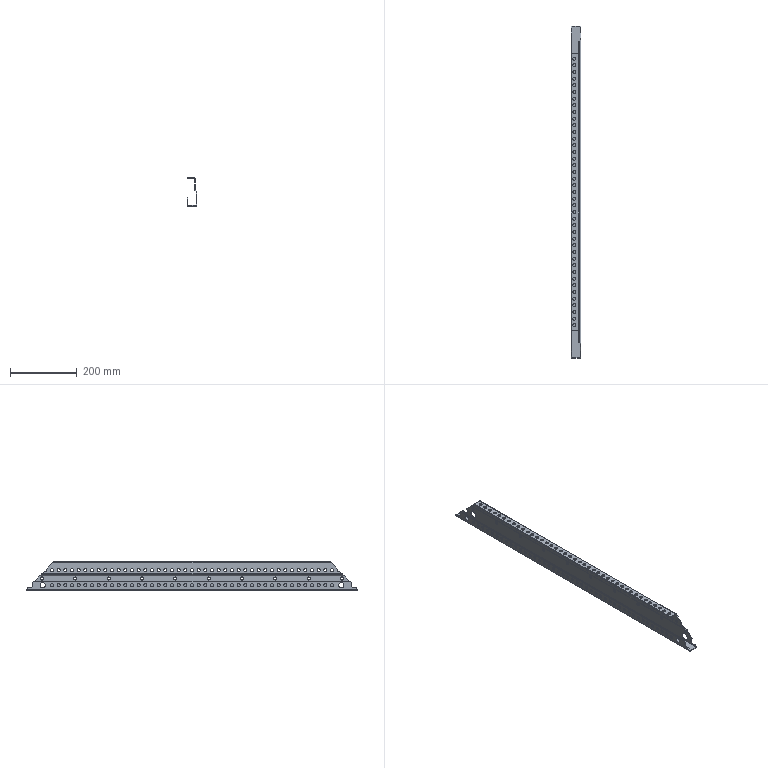Component | SolidWorks | HighVoltageCabinetFrameAssembly-1_HighVoltageCabinetHorizontalFrame-1 | 1 solid | 342 faces | volume 271676 mm3 | cylinder 300 | plane 32 | spline 10 | commonest cylinder face diameters 9.2 x277 22 x7 16 x6 1.473 x5 5.473 x5 | material Plain Carbon Steel